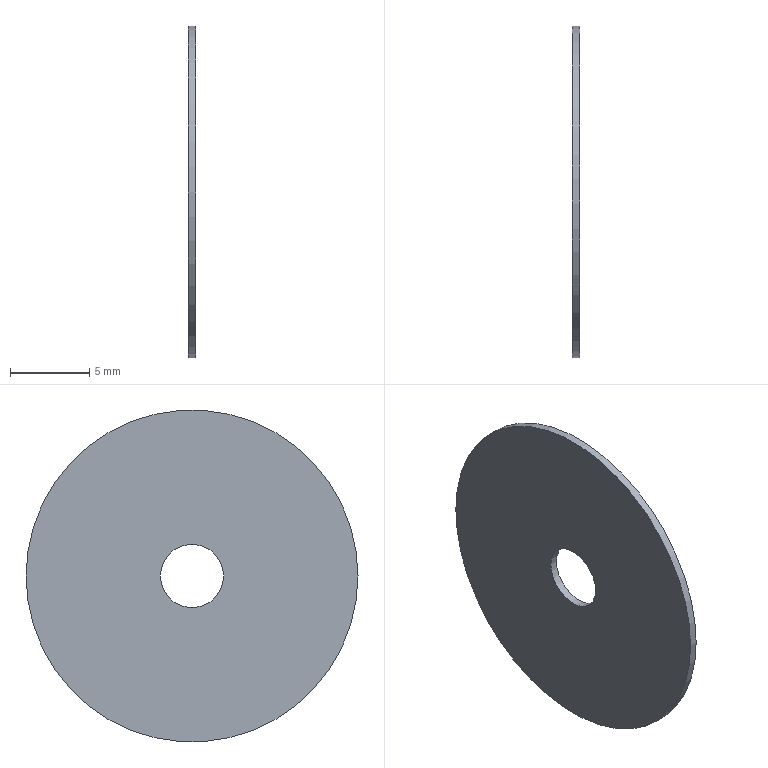Component | NX | ROUND_PLATE | 1 solid | 4 faces | volume 167 mm3 | cylinder 2 | plane 2 | commonest cylinder face diameters 21 x1 4 x1